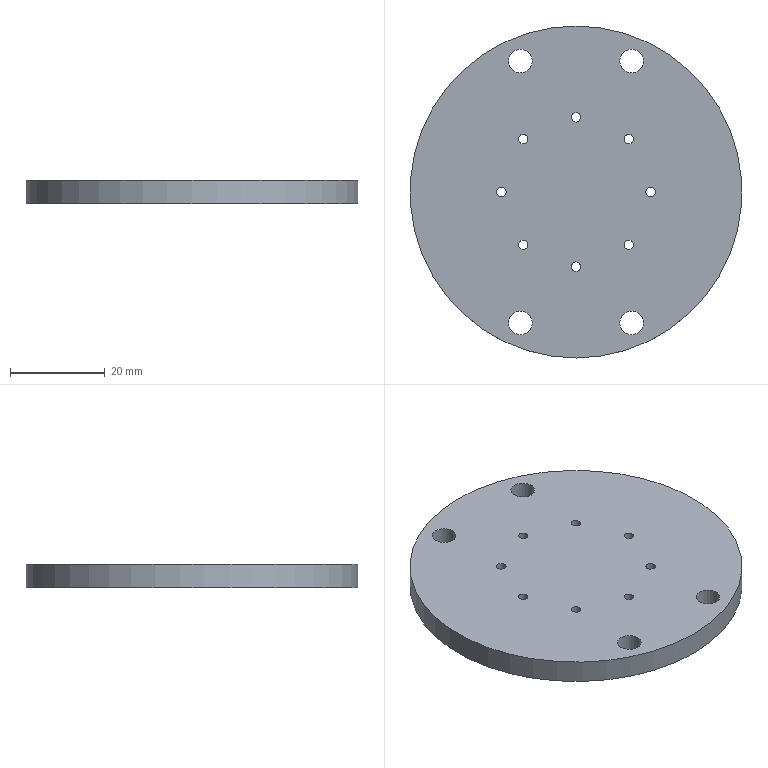Component | NX | TOPSEAT | 1 solid | 15 faces | volume 18724 mm3 | cylinder 13 | plane 2 | commonest cylinder face diameters 2 x8 5 x4 70 x1